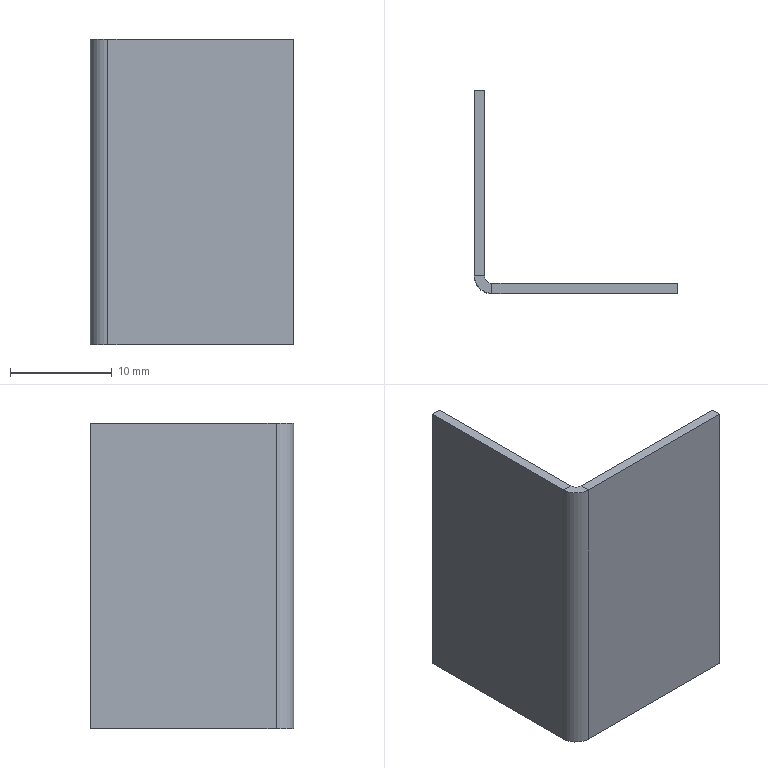Component | SolidWorks | CCQ-1.1-18Limiter-2 | 1 solid | 14 faces | volume 1154 mm3 | plane 12 | cylinder 2 | commonest cylinder face diameters 3.473 x1 1.473 x1 | material 304